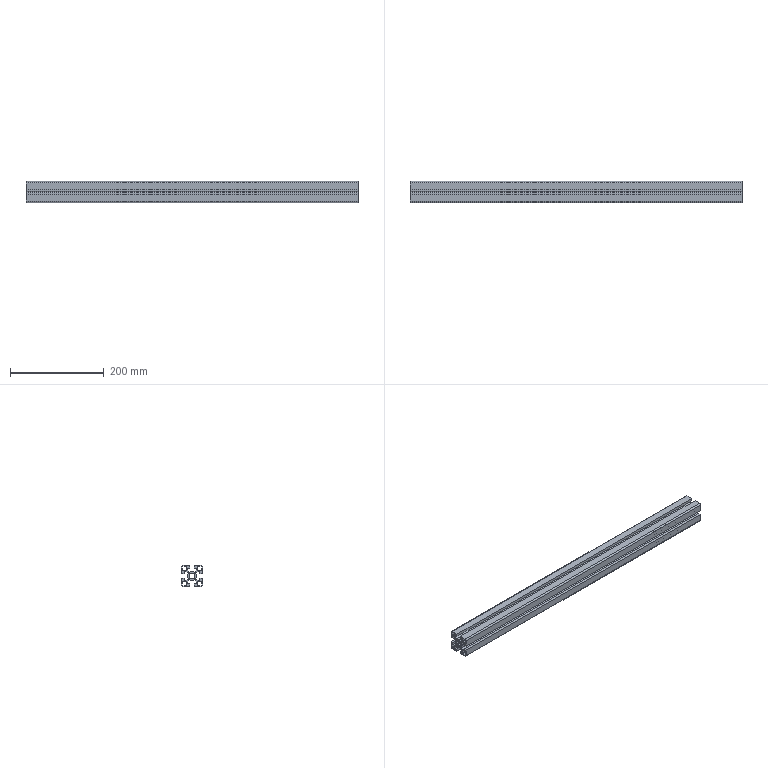Component | SolidWorks | HFS8_4545_03-B-2 | 1 solid | 131 faces | box 710 x 45 x 45 mm | volume 569562 mm3 | plane 82 | cylinder 49 | commonest cylinder face diameters 2 x18 3 x12 1 x10 12.5 x5 6 x4 | material 6061-T6 (SS)
build123d program:
from build123d import *

# Parameters (mm, degrees)
BOSS_EXTRUDE1_DEPTH = 710


with BuildPart() as part:
    # Sketch1 → Boss-Extrude1 (new body)
    with BuildSketch(Plane.XY):
        with BuildLine():
            Line((-19.5, -22.5), (-5, -22.5))
            Line((-5, -22.5), (-5, -16.5))
            Line((-5, -16.5), (-10, -16.5))
            Line((-10, -16.5), (-10, -13))
            Line((-10, -13), (-6.5, -9.5))
            Line((-6.5, -9.5), (-1.212, -9.5))
            Line((-1.212, -9.5), (0, -8.8))
            Line((0, -8.8), (1.212, -9.5))
            Line((1.212, -9.5), (6.5, -9.5))
            Line((6.5, -9.5), (10, -13))
            Line((10, -13), (10, -16.5))
            Line((10, -16.5), (5, -16.5))
            Line((5, -16.5), (5, -22.5))
            Line((5, -22.5), (19.5, -22.5))
            ThreePointArc((19.5, -22.5), (21.621, -21.621), (22.5, -19.5))
            Line((22.5, -19.5), (22.5, -5))
            Line((22.5, -5), (16.5, -5))
            Line((16.5, -5), (16.5, -10))
            Line((16.5, -10), (13, -10))
            Line((13, -10), (9.5, -6.5))
            Line((9.5, -6.5), (9.5, -1.212))
            Line((9.5, -1.212), (8.8, 0))
            Line((8.8, 0), (9.5, 1.212))
            Line((9.5, 1.212), (9.5, 6.5))
            Line((9.5, 6.5), (13, 10))
            Line((13, 10), (16.5, 10))
            Line((16.5, 10), (16.5, 5))
            Line((16.5, 5), (22.5, 5))
            Line((22.5, 5), (22.5, 19.5))
            ThreePointArc((22.5, 19.5), (21.621, 21.621), (19.5, 22.5))
            Line((19.5, 22.5), (5, 22.5))
            Line((5, 22.5), (5, 16.5))
            Line((5, 16.5), (10, 16.5))
            Line((10, 16.5), (10, 13))
            Line((10, 13), (6.5, 9.5))
            Line((6.5, 9.5), (1.212, 9.5))
            Line((1.212, 9.5), (0, 8.8))
            Line((0, 8.8), (-1.212, 9.5))
            Line((-1.212, 9.5), (-6.5, 9.5))
            Line((-6.5, 9.5), (-10, 13))
            Line((-10, 13), (-10, 16.5))
            Line((-10, 16.5), (-5, 16.5))
            Line((-5, 16.5), (-5, 22.5))
            Line((-5, 22.5), (-19.5, 22.5))
            ThreePointArc((-19.5, 22.5), (-21.621, 21.621), (-22.5, 19.5))
            Line((-22.5, 19.5), (-22.5, 5))
            Line((-22.5, 5), (-16.5, 5))
            Line((-16.5, 5), (-16.5, 10))
            Line((-16.5, 10), (-13, 10))
            Line((-13, 10), (-9.5, 6.5))
            Line((-9.5, 6.5), (-9.5, 1.212))
            Line((-9.5, 1.212), (-8.8, 0))
            Line((-8.8, 0), (-9.5, -1.212))
            Line((-9.5, -1.212), (-9.5, -6.5))
            Line((-9.5, -6.5), (-13, -10))
            Line((-13, -10), (-16.5, -10))
            Line((-16.5, -10), (-16.5, -5))
            Line((-16.5, -5), (-22.5, -5))
            Line((-22.5, -5), (-22.5, -19.5))
            ThreePointArc((-22.5, -19.5), (-21.621, -21.621), (-19.5, -22.5))
        make_face()
        with BuildLine():
            Line((12, 18.5), (12, 13))
            ThreePointArc((12, 13), (12.293, 12.293), (13, 12))
            Line((13, 12), (18.5, 12))
            ThreePointArc((18.5, 12), (19.5, 11), (20.5, 12))
            Line((20.5, 12), (20.5, 19.5))
            ThreePointArc((20.5, 19.5), (20.207, 20.207), (19.5, 20.5))
            Line((19.5, 20.5), (12, 20.5))
            ThreePointArc((12, 20.5), (11, 19.5), (12, 18.5))
        make_face(mode=Mode.SUBTRACT)
        with BuildLine():
            Line((12, -20.5), (19.5, -20.5))
            ThreePointArc((19.5, -20.5), (20.207, -20.207), (20.5, -19.5))
            Line((20.5, -19.5), (20.5, -12))
            ThreePointArc((20.5, -12), (19.5, -11), (18.5, -12))
            Line((18.5, -12), (13, -12))
            ThreePointArc((13, -12), (12.293, -12.293), (12, -13))
            Line((12, -13), (12, -18.5))
            ThreePointArc((12, -18.5), (11, -19.5), (12, -20.5))
        make_face(mode=Mode.SUBTRACT)
        with BuildLine():
            Line((-4.725, -6.139), (-3.947, -5.361))
            ThreePointArc((-3.947, -5.361), (-3.649, -5.217), (-3.327, -5.291))
            ThreePointArc((-3.327, -5.291), (0, -6.25), (3.327, -5.291))
            ThreePointArc((3.327, -5.291), (3.649, -5.217), (3.947, -5.361))
            Line((3.947, -5.361), (4.725, -6.139))
            ThreePointArc((4.725, -6.139), (7.283, -7.283), (6.139, -4.725))
            Line((6.139, -4.725), (5.361, -3.947))
            ThreePointArc((5.361, -3.947), (5.217, -3.649), (5.291, -3.327))
            ThreePointArc((5.291, -3.327), (6.25, 0), (5.291, 3.327))
            ThreePointArc((5.291, 3.327), (5.217, 3.649), (5.361, 3.947))
            Line((5.361, 3.947), (6.139, 4.725))
            ThreePointArc((6.139, 4.725), (7.283, 7.283), (4.725, 6.139))
            Line((4.725, 6.139), (3.947, 5.361))
            ThreePointArc((3.947, 5.361), (3.649, 5.217), (3.327, 5.291))
            ThreePointArc((3.327, 5.291), (0, 6.25), (-3.327, 5.291))
            ThreePointArc((-3.327, 5.291), (-3.649, 5.217), (-3.947, 5.361))
            Line((-3.947, 5.361), (-4.725, 6.139))
            ThreePointArc((-4.725, 6.139), (-7.283, 7.283), (-6.139, 4.725))
            Line((-6.139, 4.725), (-5.361, 3.947))
            ThreePointArc((-5.361, 3.947), (-5.217, 3.649), (-5.291, 3.327))
            ThreePointArc((-5.291, 3.327), (-6.25, 0), (-5.291, -3.327))
            ThreePointArc((-5.291, -3.327), (-5.217, -3.649), (-5.361, -3.947))
            Line((-5.361, -3.947), (-6.139, -4.725))
            ThreePointArc((-6.139, -4.725), (-7.283, -7.283), (-4.725, -6.139))
        make_face(mode=Mode.SUBTRACT)
        with BuildLine():
            Line((-19.5, -20.5), (-12, -20.5))
            ThreePointArc((-12, -20.5), (-11, -19.5), (-12, -18.5))
            Line((-12, -18.5), (-12, -13))
            ThreePointArc((-12, -13), (-12.293, -12.293), (-13, -12))
            Line((-13, -12), (-18.5, -12))
            ThreePointArc((-18.5, -12), (-19.5, -11), (-20.5, -12))
            Line((-20.5, -12), (-20.5, -19.5))
            ThreePointArc((-20.5, -19.5), (-20.207, -20.207), (-19.5, -20.5))
        make_face(mode=Mode.SUBTRACT)
        with BuildLine():
            Line((-18.5, 12), (-13, 12))
            ThreePointArc((-13, 12), (-12.293, 12.293), (-12, 13))
            Line((-12, 13), (-12, 18.5))
            ThreePointArc((-12, 18.5), (-11, 19.5), (-12, 20.5))
            Line((-12, 20.5), (-19.5, 20.5))
            ThreePointArc((-19.5, 20.5), (-20.207, 20.207), (-20.5, 19.5))
            Line((-20.5, 19.5), (-20.5, 12))
            ThreePointArc((-20.5, 12), (-19.5, 11), (-18.5, 12))
        make_face(mode=Mode.SUBTRACT)
    extrude(amount=-BOSS_EXTRUDE1_DEPTH)


solid = part.part

# Placed as in the assembly
solid = solid.moved(Location((-88.006, 8.087, -2380.428), (0, 90, 0)))